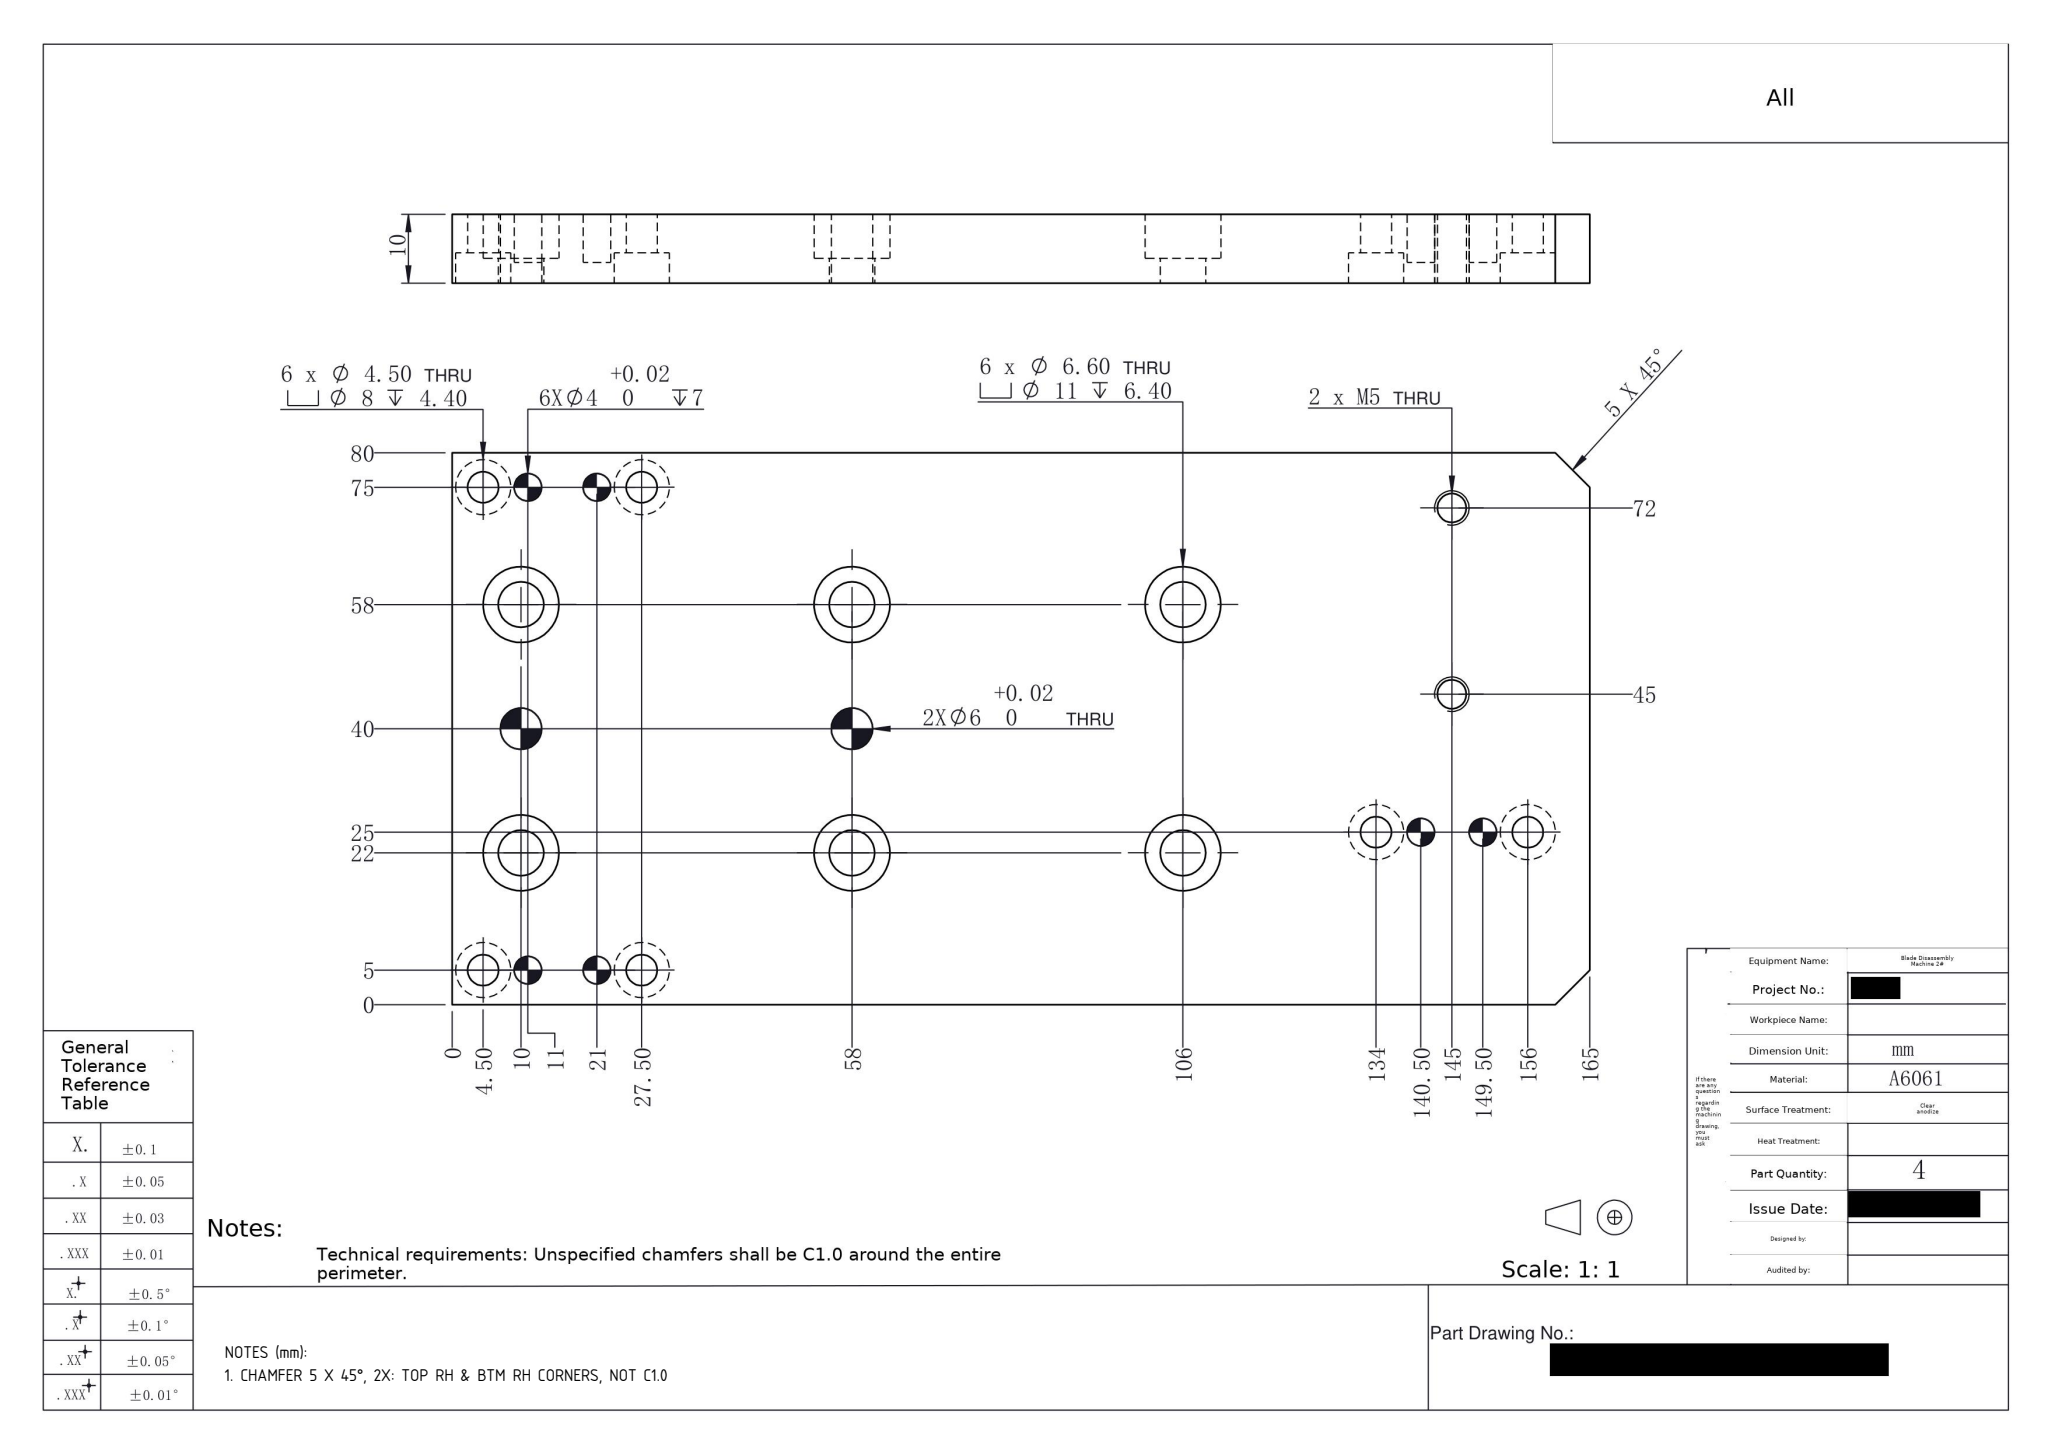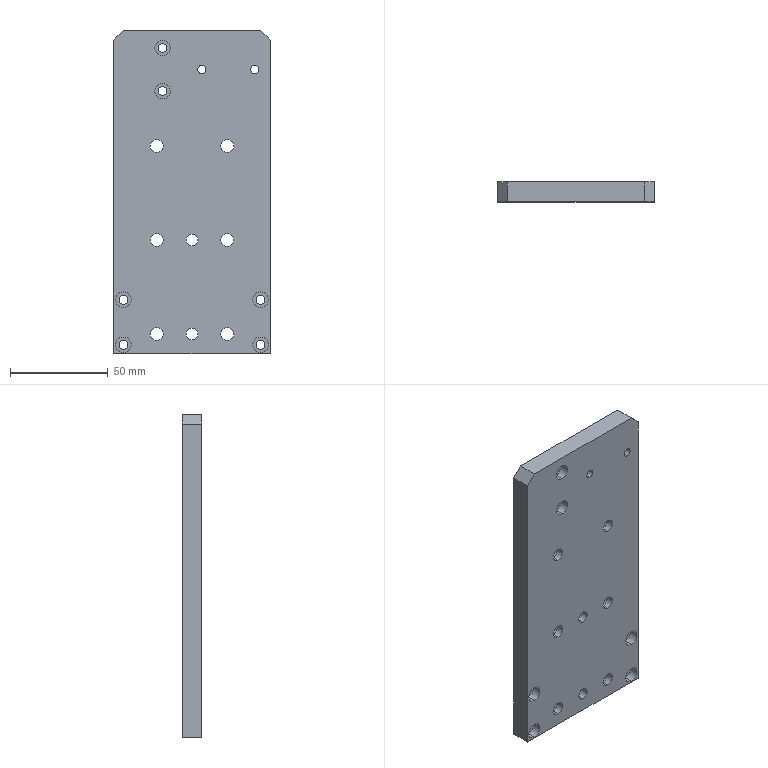Part | SolidWorks | mm | 1 solid | 94 faces | box 80 x 10 x 165 mm | volume 124130 mm3 | cylinder 68 | plane 26 | commonest cylinder face diameters 11 x12 6.6 x12 4 x12 8 x12 4.5 x12 4.2 x4 6 x4
Drawing notes:
CHAMFER 5 X 45°, 2X: TOP RH & BTM RH CORNERS, NOT C1.0 | from the solid: Model bbox 165 x 80 x 10, no fillet radii; planar corner cuts match 5 X 45 deg callout, mirrored about 40 CL
build123d program:
from build123d import *

# Parameters (mm, degrees)
SKETCH1_W                                       = 80
SKETCH1_H                                       = 165
BOSS_EXTRUDE1_DEPTH                             = 5
M4_HEX_SOCKET_HEAD_CAP_SCREW_CBORE1_D           = 4.5
M4_HEX_SOCKET_HEAD_CAP_SCREW_CBORE1_CBORE_D     = 8
M4_HEX_SOCKET_HEAD_CAP_SCREW_CBORE1_CBORE_DEPTH = 4.4
F_4_0MM_DOWEL_PIN_HOLE1_D                       = 4
F_4_0MM_DOWEL_PIN_HOLE1_DEPTH                   = 7
CHAMFER1_SIZE                                   = 5
M6_HEX_SOCKET_HEAD_CAP_SCREW_CBORE1_D           = 6.6
M6_HEX_SOCKET_HEAD_CAP_SCREW_CBORE1_CBORE_D     = 11
M6_HEX_SOCKET_HEAD_CAP_SCREW_CBORE1_CBORE_DEPTH = 6.4
F_6_0MM_DOWEL_PIN_HOLE1_D                       = 6
M5_TAPPED_HOLE1_D                               = 4.2


with BuildPart() as part:
    # Sketch1 → Boss-Extrude1 (new, symmetric)
    with BuildSketch(Plane(origin=(0, 0, 0), x_dir=(1, 0, 0), z_dir=(0, 1, 0))):
        Rectangle(SKETCH1_W, SKETCH1_H)
    extrude(amount=BOSS_EXTRUDE1_DEPTH, both=True)

    # M4 Hex Socket Head Cap Screw CBORE1 (through all)
    with Locations(Plane(origin=(0, -5, 0), x_dir=(-1, 0, 0), z_dir=(0, -1, 0))):
        with Locations((-35, 78), (-35, 55), (35, 78), (35, 55), (15, -51.5), (15, -73.5)):
            CounterBoreHole(M4_HEX_SOCKET_HEAD_CAP_SCREW_CBORE1_D / 2, M4_HEX_SOCKET_HEAD_CAP_SCREW_CBORE1_CBORE_D / 2, M4_HEX_SOCKET_HEAD_CAP_SCREW_CBORE1_CBORE_DEPTH)

    # 4.0mm Dowel Pin Hole1
    with Locations(Plane(origin=(0, 5, 0), x_dir=(1, 0, 0), z_dir=(0, 1, 0))):
        with Locations((-15, -58), (-15, -67), (-35, 71.5), (-35, 61.5), (35, 71.5), (35, 61.5)):
            Hole(F_4_0MM_DOWEL_PIN_HOLE1_D / 2, depth=F_4_0MM_DOWEL_PIN_HOLE1_DEPTH)

    # Chamfer1
    chamfer1_edges = [part.edges().sort_by_distance(p)[0] for p in [
        (40, 0, 82.5),
        (-40, 0, 82.5),
    ]]
    chamfer(chamfer1_edges, length=CHAMFER1_SIZE)

    # M6 Hex Socket Head Cap Screw CBORE1 (through all)
    with Locations(Plane(origin=(0, 5, 0), x_dir=(1, 0, 0), z_dir=(0, 1, 0))):
        with Locations((-18, 72.5), (18, 72.5), (18, 24.5), (-18, 24.5), (-18, -23.5), (18, -23.5)):
            CounterBoreHole(M6_HEX_SOCKET_HEAD_CAP_SCREW_CBORE1_D / 2, M6_HEX_SOCKET_HEAD_CAP_SCREW_CBORE1_CBORE_D / 2, M6_HEX_SOCKET_HEAD_CAP_SCREW_CBORE1_CBORE_DEPTH)

    # 6.0mm Dowel Pin Hole1 (through all)
    with Locations(Plane(origin=(0, 5, 0), x_dir=(1, 0, 0), z_dir=(0, 1, 0))):
        with Locations((0, 72.5), (0, 24.5)):
            Hole(F_6_0MM_DOWEL_PIN_HOLE1_D / 2)

    # M5 Tapped Hole1 (through all)
    with Locations(Plane(origin=(0, 5, 0), x_dir=(1, 0, 0), z_dir=(0, 1, 0))):
        with Locations((5, -62.5), (32, -62.5)):
            Hole(M5_TAPPED_HOLE1_D / 2)


solid = part.part